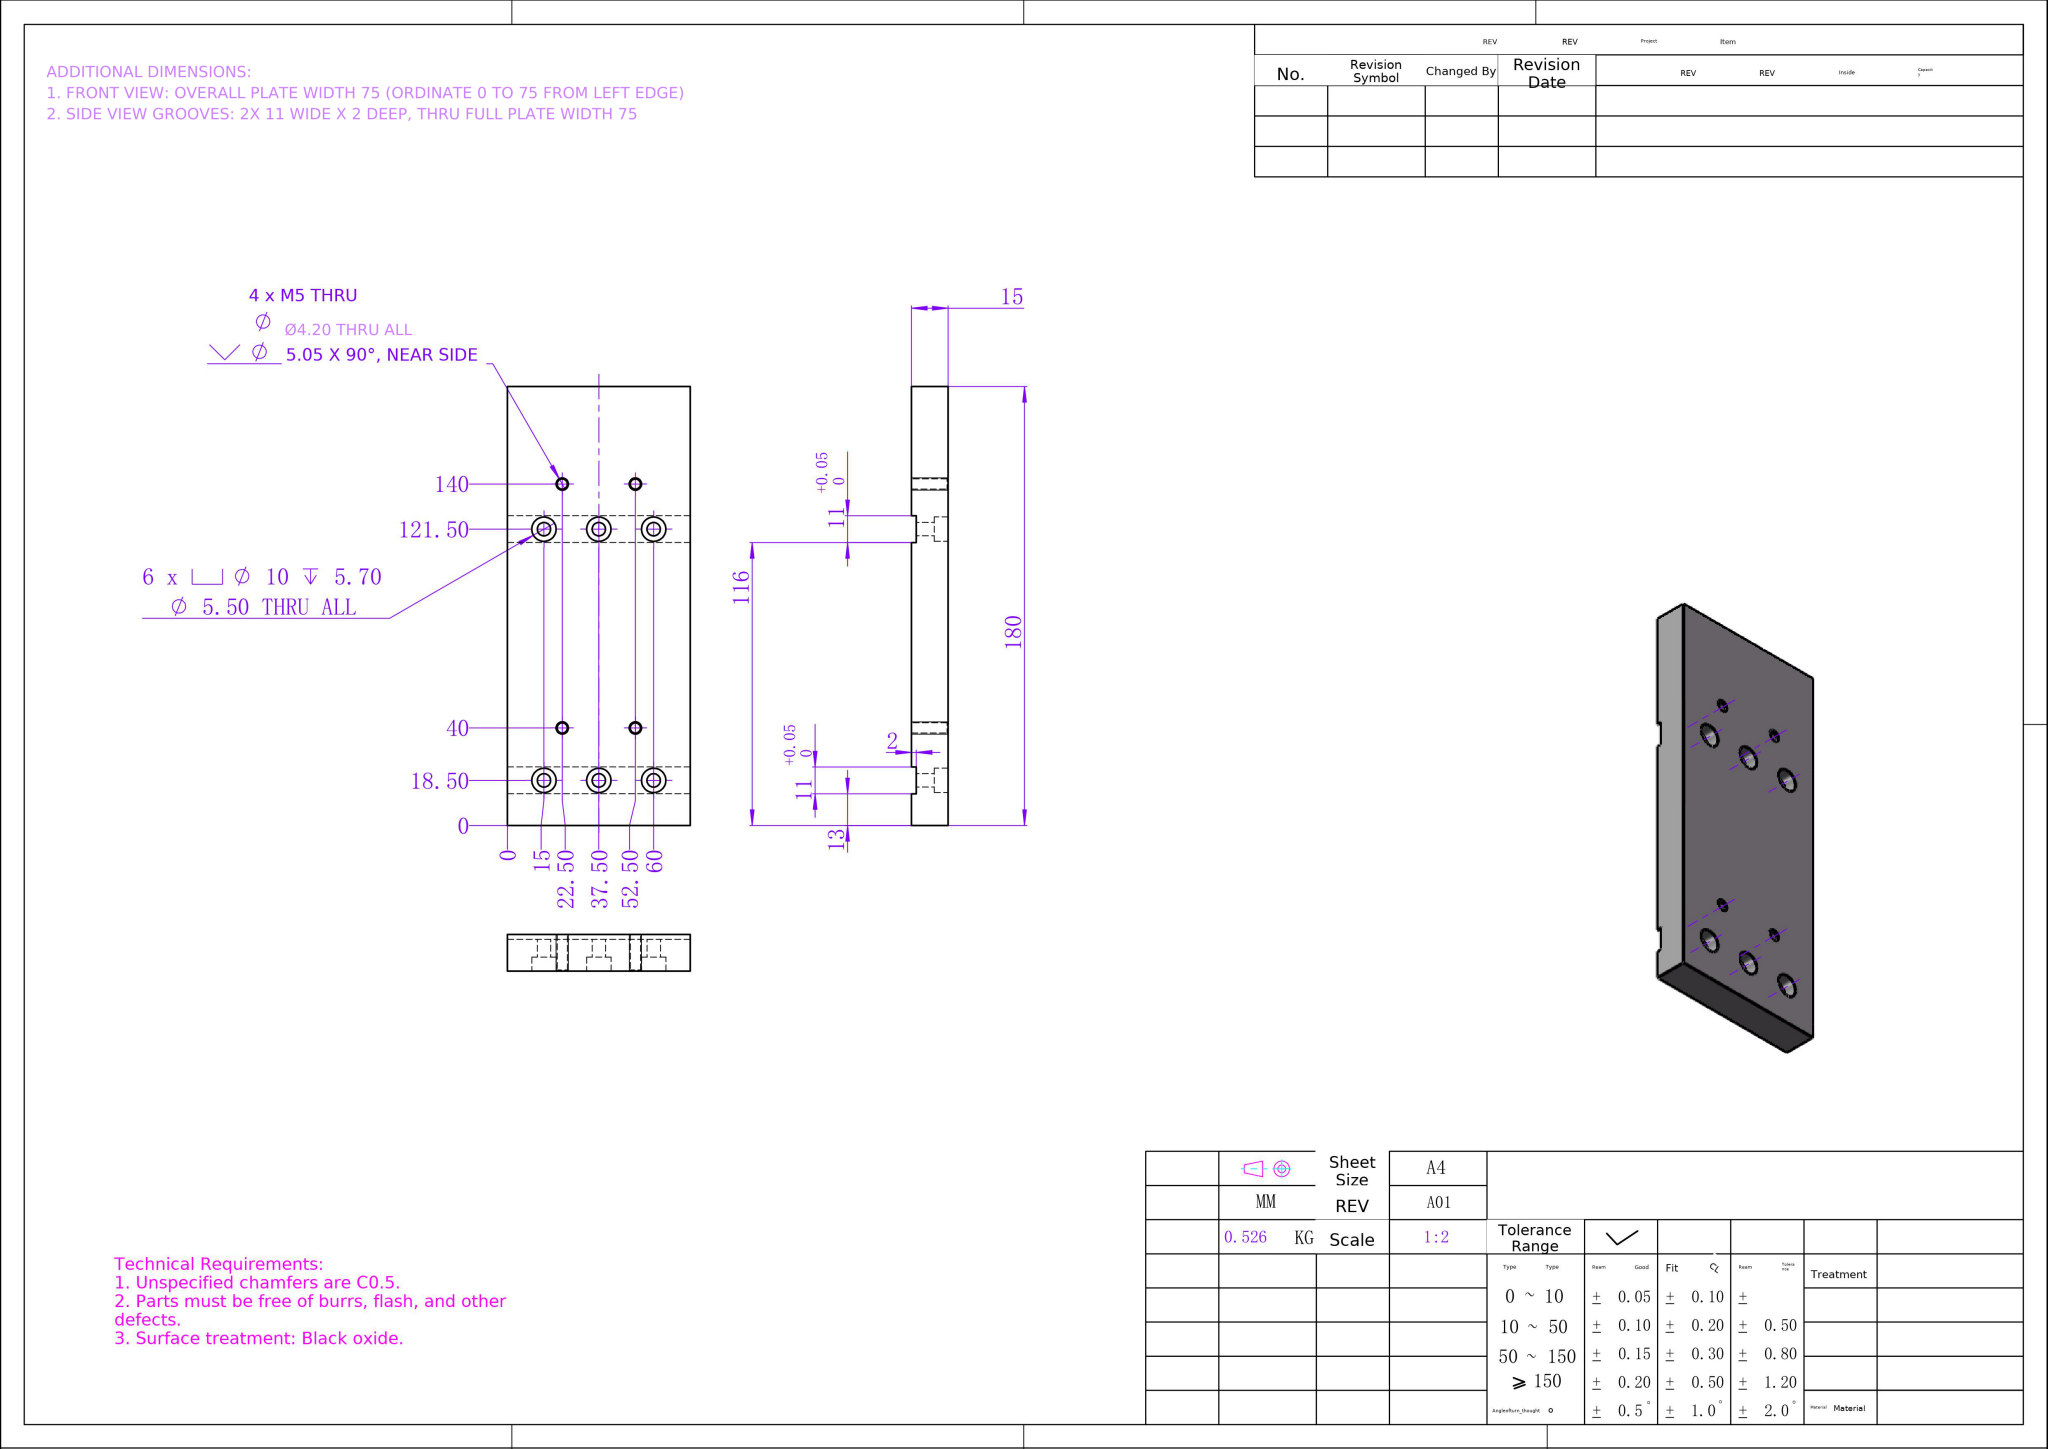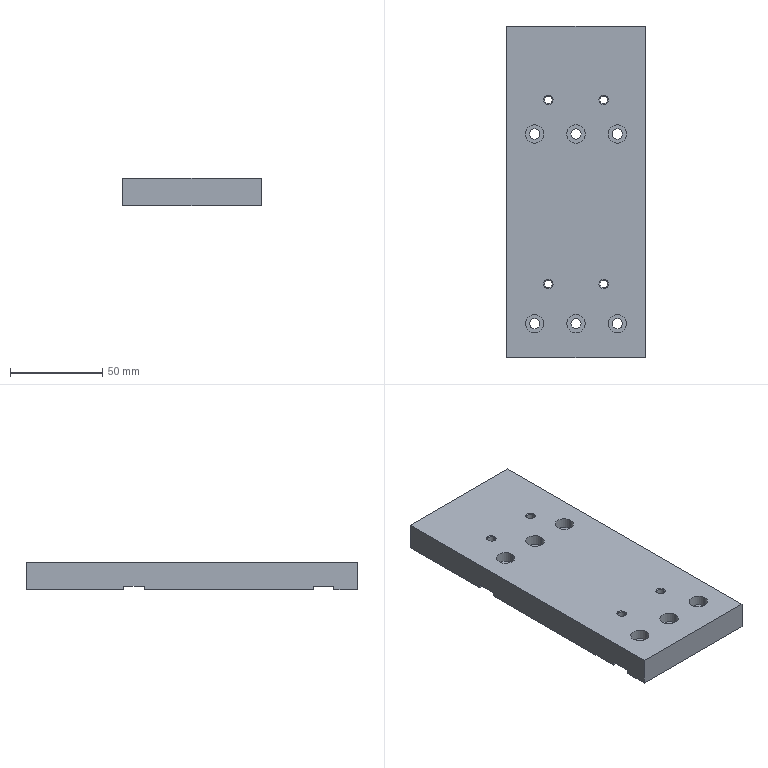Part | NX | mm | 1 solid | 60 faces | box 75 x 180 x 15 mm | volume 194637 mm3 | cylinder 32 | plane 20 | cone 8 | commonest cylinder face diameters 10 x12 5.5 x12 4.2 x8